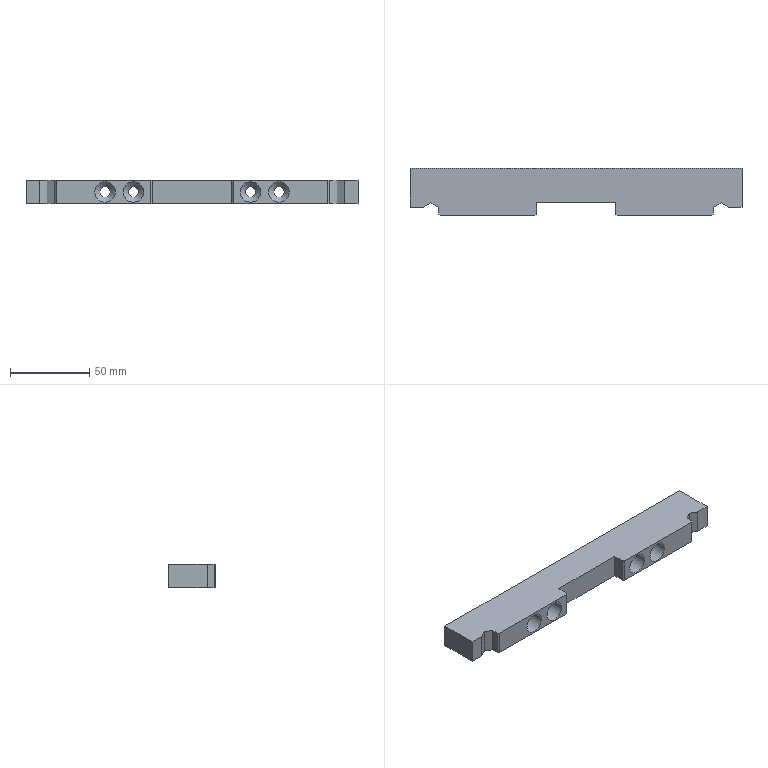Component | SolidWorks | YS01-071NozzleFasteningClampBlock-1 | 1 solid | 46 faces | box 210 x 29.95 x 15 mm | volume 74377 mm3 | plane 22 | cylinder 16 | cone 8 | commonest cylinder face diameters 6.6 x8 13 x8
build123d program:
from build123d import *

# Parameters (mm, degrees)
BOSS_EXTRUDE1_DEPTH                                  = 15
SKETCH2_W                                            = 50
SKETCH2_H                                            = 16.2
CUT_EXTRUDE1_DEPTH                                   = 124.048
CHAMFER1_SIZE                                        = 1
SKETCH4_W                                            = 15
SKETCH4_H                                            = 24.598
BOSS_EXTRUDE2_DEPTH                                  = 8.45
SKETCH5_W                                            = 15
SKETCH5_H                                            = 24.598
BOSS_EXTRUDE3_DEPTH                                  = 8.45
SKETCH9_R                                            = 6.5
CUT_EXTRUDE3_DEPTH                                   = 15
M6_HEX_SOCKET_COUNTERSUNK_HEAD_SCREW_COU_D           = 6.6
M6_HEX_SOCKET_COUNTERSUNK_HEAD_SCREW_COU_CSINK_D     = 13
M6_HEX_SOCKET_COUNTERSUNK_HEAD_SCREW_COU_CSINK_ANGLE = 90


with BuildPart() as part:
    # Sketch1 → Boss-Extrude1 (new body)
    with BuildSketch(Plane.XY):
        Polygon((-74.05, 2.66), (-74.05, 27.258), (119.05, 27.258), (119.05, 2.66), (114.3, 5.402), (109.45, 2.602), (109.45, -2.692), (-64.45, -2.692), (-64.45, 2.602), (-69.3, 5.402), align=None)
    extrude(amount=-BOSS_EXTRUDE1_DEPTH)

    # Sketch2 → Cut-Extrude1 (cut, through all)
    with BuildSketch(Plane.XY):
        with Locations((22.5, -2.692)):
            Rectangle(SKETCH2_W, SKETCH2_H)
    extrude(amount=-CUT_EXTRUDE1_DEPTH, mode=Mode.SUBTRACT)

    # Chamfer1
    chamfer1_edges = [part.edges().sort_by_distance(p)[0] for p in [
        (-64.45, -2.692, -7.5),
        (109.45, -2.692, -7.5),
        (47.5, -2.692, -7.5),
        (-2.5, -2.692, -7.5),
    ]]
    chamfer(chamfer1_edges, length=CHAMFER1_SIZE)

    # Sketch4 → Boss-Extrude2 (add)
    with BuildSketch(Plane.ZY.offset(74.05)):
        with Locations((-7.5, 14.959)):
            Rectangle(SKETCH4_W, SKETCH4_H)
    extrude(amount=BOSS_EXTRUDE2_DEPTH)

    # Sketch5 → Boss-Extrude3 (add)
    with BuildSketch(Plane(origin=(119.05, 0, 0), x_dir=(0, 0, -1), z_dir=(1, 0, 0))):
        with Locations((7.5, 14.959)):
            Rectangle(SKETCH5_W, SKETCH5_H)
    extrude(amount=BOSS_EXTRUDE3_DEPTH)

    # Sketch9 → Cut-Extrude3 (cut)
    with BuildSketch(Plane(origin=(0, -2.692, 0), x_dir=(-1, 0, 0), z_dir=(0, -1, 0))):
        with Locations(Location((-77.5, 7.5, 0), (0, 0, 180))):
            Circle(SKETCH9_R)
        with Locations(Location((-59.5, 7.5, 0), (0, 0, 180))):
            Circle(SKETCH9_R)
    cut_extrude3 = extrude(amount=-CUT_EXTRUDE3_DEPTH, mode=Mode.SUBTRACT)

    # M6 Hex Socket Countersunk Head Screw Cou (through all)
    with Locations(Plane(origin=(0, 12.308, 0), x_dir=(-1, 0, 0), z_dir=(0, -1, 0))):
        with Locations((-77.5, 7.5), (-59.5, 7.5)):
            m6_hex_socket_countersunk_head_screw_cou = CounterSinkHole(M6_HEX_SOCKET_COUNTERSUNK_HEAD_SCREW_COU_D / 2, M6_HEX_SOCKET_COUNTERSUNK_HEAD_SCREW_COU_CSINK_D / 2, counter_sink_angle=M6_HEX_SOCKET_COUNTERSUNK_HEAD_SCREW_COU_CSINK_ANGLE)

    # Mirror1: Cut-Extrude3, M6 Hex Socket Countersunk Head Screw Cou across plane
    add(cut_extrude3.mirror(Plane(origin=(22.5, 0, 0), x_dir=(0, 0, 1), z_dir=(1, 0, 0))), mode=Mode.SUBTRACT)
    add(m6_hex_socket_countersunk_head_screw_cou.mirror(Plane(origin=(22.5, 0, 0), x_dir=(0, 0, 1), z_dir=(1, 0, 0))), mode=Mode.SUBTRACT)


solid = part.part

# Placed as in the assembly
solid = solid.moved(Location((-589.112, -348.131, 2414.9), (0, 0, 0)))